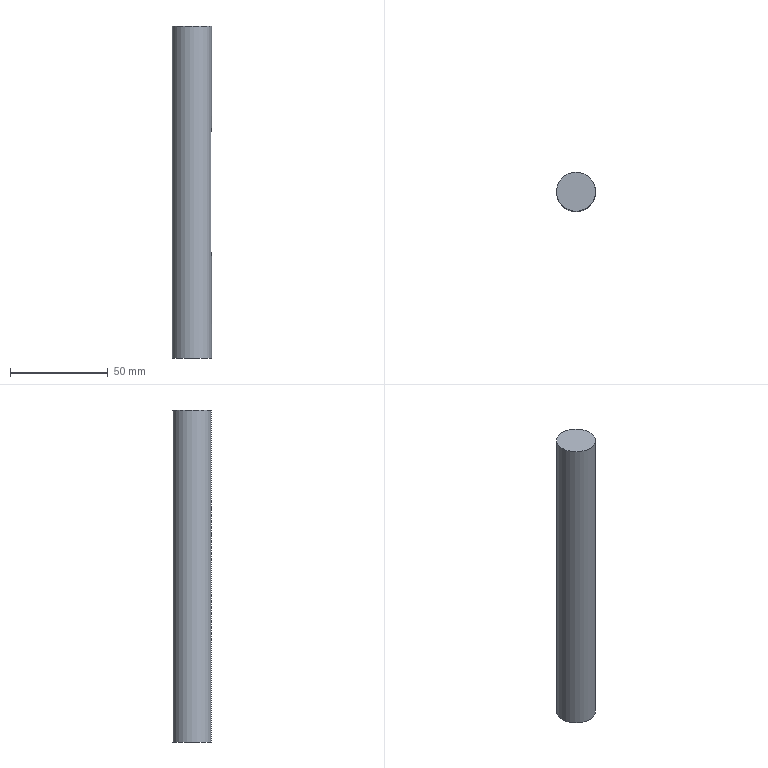Component | NX | CAMSHAFT | 1 solid | 8 faces | box 20 x 20 x 170 mm | volume 52641 mm3 | plane 5 | cylinder 3 | commonest cylinder face diameters 5 x2 20 x1
STEP:
#1=CARTESIAN_POINT('',(0.,0.,0.));
#2=DIRECTION('',(0.,0.,1.));
#3=DIRECTION('',(1.,0.,0.));
#4=AXIS2_PLACEMENT_3D('',#1,#2,#3);
#5=CARTESIAN_POINT('',(10.,0.,90.));
#6=VERTEX_POINT('',#5);
#7=CARTESIAN_POINT('',(0.,0.,90.));
#8=DIRECTION('',(0.,0.,1.));
#9=DIRECTION('',(1.,0.,0.));
#10=AXIS2_PLACEMENT_3D('',#7,#8,#9);
#11=CIRCLE('',#10,10.);
#12=CARTESIAN_POINT('',(0.,0.,260.));
#13=DIRECTION('',(0.,0.,-1.));
#14=DIRECTION('',(-1.,0.,0.));
#15=AXIS2_PLACEMENT_3D('',#12,#13,#14);
#16=CYLINDRICAL_SURFACE('',#15,10.);
#17=CARTESIAN_POINT('',(9.425,170.));
#18=DIRECTION('',(-1.,0.));
#19=VECTOR('',#18,1.);
#20=LINE('',#17,#19);
#21=(GEOMETRIC_REPRESENTATION_CONTEXT(2)PARAMETRIC_REPRESENTATION_CONTEXT()REPRESENTATION_CONTEXT('',''));
#22=DEFINITIONAL_REPRESENTATION('',(#20),#21);
#23=PCURVE('',#16,#22);
#24=CARTESIAN_POINT('',(0.,0.,90.));
#25=DIRECTION('',(0.,0.,1.));
#26=DIRECTION('',(1.,0.,0.));
#27=AXIS2_PLACEMENT_3D('',#24,#25,#26);
#28=PLANE('',#27);
#29=CARTESIAN_POINT('',(0.,0.));
#30=DIRECTION('',(1.,0.));
#31=AXIS2_PLACEMENT_2D('',#29,#30);
#32=CIRCLE('',#31,10.);
#33=(GEOMETRIC_REPRESENTATION_CONTEXT(2)PARAMETRIC_REPRESENTATION_CONTEXT()REPRESENTATION_CONTEXT('',''));
#34=DEFINITIONAL_REPRESENTATION('',(#32),#33);
#35=PCURVE('',#28,#34);
#36=SURFACE_CURVE('',#11,(#23,#35),.PCURVE_S1.);
#37=EDGE_CURVE('',#6,#6,#36,.T.);
#38=ORIENTED_EDGE('',*,*,#37,.T.);
#39=CARTESIAN_POINT('',(10.,0.,142.5));
#40=VERTEX_POINT('',#39);
#41=CARTESIAN_POINT('',(10.,0.,142.5));
#42=CARTESIAN_POINT('',(10.,0.,90.));
#43=B_SPLINE_CURVE_WITH_KNOTS('',1,(#41,#42),.UNSPECIFIED.,.F.,.F.,(2,2),(117.5,170.),.PIECEWISE_BEZIER_KNOTS.);
#44=CARTESIAN_POINT('',(3.142,0.));
#45=DIRECTION('',(0.,1.));
#46=VECTOR('',#45,1.);
#47=LINE('',#44,#46);
#48=(GEOMETRIC_REPRESENTATION_CONTEXT(2)PARAMETRIC_REPRESENTATION_CONTEXT()REPRESENTATION_CONTEXT('',''));
#49=DEFINITIONAL_REPRESENTATION('',(#47),#48);
#50=PCURVE('',#16,#49);
#51=CARTESIAN_POINT('',(9.425,0.));
#52=DIRECTION('',(0.,1.));
#53=VECTOR('',#52,1.);
#54=LINE('',#51,#53);
#55=(GEOMETRIC_REPRESENTATION_CONTEXT(2)PARAMETRIC_REPRESENTATION_CONTEXT()REPRESENTATION_CONTEXT('',''));
#56=DEFINITIONAL_REPRESENTATION('',(#54),#55);
#57=PCURVE('',#16,#56);
#58=SEAM_CURVE('',#43,(#50,#57),.PCURVE_S1.);
#59=EDGE_CURVE('',#40,#6,#58,.T.);
#60=ORIENTED_EDGE('',*,*,#59,.F.);
#61=CARTESIAN_POINT('',(9.682,-2.5,145.));
#62=VERTEX_POINT('',#61);
#63=CARTESIAN_POINT('',(9.682,-2.5,145.));
#64=CARTESIAN_POINT('',(9.682,-2.5,144.725));
#65=CARTESIAN_POINT('',(9.695,-2.453,144.446));
#66=CARTESIAN_POINT('',(9.717,-2.364,144.187));
#67=CARTESIAN_POINT('',(9.738,-2.275,143.928));
#68=CARTESIAN_POINT('',(9.769,-2.142,143.682));
#69=CARTESIAN_POINT('',(9.803,-1.974,143.466));
#70=CARTESIAN_POINT('',(9.838,-1.804,143.247));
#71=CARTESIAN_POINT('',(9.875,-1.594,143.054));
#72=CARTESIAN_POINT('',(9.907,-1.36,142.902));
#73=CARTESIAN_POINT('',(9.94,-1.123,142.749));
#74=CARTESIAN_POINT('',(9.967,-0.8559,142.634));
#75=CARTESIAN_POINT('',(9.983,-0.5801,142.568));
#76=CARTESIAN_POINT('',(9.999,-0.31,142.504));
#77=CARTESIAN_POINT('',(10.004,-0.02421,142.485));
#78=CARTESIAN_POINT('',(9.997,0.2525,142.513));
#79=CARTESIAN_POINT('',(9.99,0.523,142.54));
#80=CARTESIAN_POINT('',(9.972,0.7923,142.613));
#81=CARTESIAN_POINT('',(9.946,1.039,142.726));
#82=CARTESIAN_POINT('',(9.92,1.287,142.84));
#83=CARTESIAN_POINT('',(9.886,1.519,142.996));
#84=CARTESIAN_POINT('',(9.851,1.717,143.183));
#85=CARTESIAN_POINT('',(9.816,1.921,143.375));
#86=CARTESIAN_POINT('',(9.779,2.094,143.605));
#87=CARTESIAN_POINT('',(9.75,2.222,143.854));
#88=CARTESIAN_POINT('',(9.721,2.351,144.105));
#89=CARTESIAN_POINT('',(9.698,2.439,144.382));
#90=CARTESIAN_POINT('',(9.688,2.477,144.663));
#91=CARTESIAN_POINT('',(9.684,2.492,144.774));
#92=CARTESIAN_POINT('',(9.682,2.5,144.887));
#93=CARTESIAN_POINT('',(9.682,2.5,145.));
#94=B_SPLINE_CURVE_WITH_KNOTS('',3,(#63,#64,#65,#66,#67,#68,#69,#70,#71,#72,#73,#74,#75,#76,#77,#78,#79,#80,#81,#82,#83,#84,#85,#86,#87,#88,#89,#90,#91,#92,#93),.UNSPECIFIED.,.F.,.F.,(4,3,3,3,3,3,3,3,3,3,4),(0.,0.1051,0.2101,0.3172,0.4259,0.5323,0.6363,0.7412,0.849,0.9574,1.),.UNSPECIFIED.);
#95=CARTESIAN_POINT('',(3.394,115.));
#96=CARTESIAN_POINT('',(3.394,115.059));
#97=CARTESIAN_POINT('',(3.394,115.179));
#98=CARTESIAN_POINT('',(3.392,115.357));
#99=CARTESIAN_POINT('',(3.389,115.534));
#100=CARTESIAN_POINT('',(3.384,115.707));
#101=CARTESIAN_POINT('',(3.378,115.876));
#102=CARTESIAN_POINT('',(3.371,116.041));
#103=CARTESIAN_POINT('',(3.363,116.201));
#104=CARTESIAN_POINT('',(3.354,116.354));
#105=CARTESIAN_POINT('',(3.343,116.5));
#106=CARTESIAN_POINT('',(3.332,116.638));
#107=CARTESIAN_POINT('',(3.319,116.769));
#108=CARTESIAN_POINT('',(3.306,116.89));
#109=CARTESIAN_POINT('',(3.292,117.002));
#110=CARTESIAN_POINT('',(3.277,117.104));
#111=CARTESIAN_POINT('',(3.262,117.194));
#112=CARTESIAN_POINT('',(3.246,117.274));
#113=CARTESIAN_POINT('',(3.229,117.343));
#114=CARTESIAN_POINT('',(3.212,117.4));
#115=CARTESIAN_POINT('',(3.195,117.444));
#116=CARTESIAN_POINT('',(3.178,117.476));
#117=CARTESIAN_POINT('',(3.16,117.495));
#118=CARTESIAN_POINT('',(3.142,117.502));
#119=CARTESIAN_POINT('',(3.124,117.496));
#120=CARTESIAN_POINT('',(3.106,117.477));
#121=CARTESIAN_POINT('',(3.088,117.445));
#122=CARTESIAN_POINT('',(3.071,117.4));
#123=CARTESIAN_POINT('',(3.054,117.344));
#124=CARTESIAN_POINT('',(3.037,117.276));
#125=CARTESIAN_POINT('',(3.021,117.196));
#126=CARTESIAN_POINT('',(3.006,117.105));
#127=CARTESIAN_POINT('',(2.991,117.003));
#128=CARTESIAN_POINT('',(2.977,116.891));
#129=CARTESIAN_POINT('',(2.964,116.771));
#130=CARTESIAN_POINT('',(2.952,116.64));
#131=CARTESIAN_POINT('',(2.94,116.502));
#132=CARTESIAN_POINT('',(2.93,116.355));
#133=CARTESIAN_POINT('',(2.92,116.202));
#134=CARTESIAN_POINT('',(2.912,116.044));
#135=CARTESIAN_POINT('',(2.905,115.879));
#136=CARTESIAN_POINT('',(2.899,115.709));
#137=CARTESIAN_POINT('',(2.895,115.535));
#138=CARTESIAN_POINT('',(2.891,115.36));
#139=CARTESIAN_POINT('',(2.889,115.181));
#140=CARTESIAN_POINT('',(2.889,115.06));
#141=CARTESIAN_POINT('',(2.889,115.));
#142=B_SPLINE_CURVE_WITH_KNOTS('',3,(#95,#96,#97,#98,#99,#100,#101,#102,#103,#104,#105,#106,#107,#108,#109,#110,#111,#112,#113,#114,#115,#116,#117,#118,#119,#120,#121,#122,#123,#124,#125,#126,#127,#128,#129,#130,#131,#132,#133,#134,#135,#136,#137,#138,#139,#140,#141),.UNSPECIFIED.,.F.,.F.,(4,1,1,1,1,1,1,1,1,1,1,1,1,1,1,1,1,1,1,1,1,1,1,1,1,1,1,1,1,1,1,1,1,1,1,1,1,1,1,1,1,1,1,1,4),(0.,0.02273,0.04545,0.06818,0.09091,0.1136,0.1364,0.1591,0.1818,0.2045,0.2273,0.25,0.2727,0.2955,0.3182,0.3409,0.3636,0.3864,0.4091,0.4318,0.4545,0.4773,0.5,0.5227,0.5455,0.5682,0.5909,0.6136,0.6364,0.6591,0.6818,0.7045,0.7273,0.75,0.7727,0.7955,0.8182,0.8409,0.8636,0.8864,0.9091,0.9318,0.9545,0.9773,1.),.QUASI_UNIFORM_KNOTS.);
#143=(GEOMETRIC_REPRESENTATION_CONTEXT(2)PARAMETRIC_REPRESENTATION_CONTEXT()REPRESENTATION_CONTEXT('',''));
#144=DEFINITIONAL_REPRESENTATION('',(#142),#143);
#145=PCURVE('',#16,#144);
#146=CARTESIAN_POINT('',(32.,0.,145.));
#147=DIRECTION('',(-1.,0.,0.));
#148=DIRECTION('',(0.,0.,1.));
#149=AXIS2_PLACEMENT_3D('',#146,#147,#148);
#150=CYLINDRICAL_SURFACE('',#149,2.5);
#151=CARTESIAN_POINT('',(4.712,22.318));
#152=CARTESIAN_POINT('',(3.142,22.));
#153=B_SPLINE_CURVE_WITH_KNOTS('',1,(#151,#152),.UNSPECIFIED.,.F.,.F.,(2,2),(0.,0.5001),.PIECEWISE_BEZIER_KNOTS.);
#154=(GEOMETRIC_REPRESENTATION_CONTEXT(2)PARAMETRIC_REPRESENTATION_CONTEXT()REPRESENTATION_CONTEXT('',''));
#155=DEFINITIONAL_REPRESENTATION('',(#153),#154);
#156=PCURVE('',#150,#155);
#157=SURFACE_CURVE('',#94,(#145,#156),.PCURVE_S1.);
#158=EDGE_CURVE('',#62,#40,#157,.T.);
#159=ORIENTED_EDGE('',*,*,#158,.F.);
#160=CARTESIAN_POINT('',(9.682,-2.5,205.));
#161=VERTEX_POINT('',#160);
#162=CARTESIAN_POINT('',(9.682,-2.5,260.));
#163=DIRECTION('',(0.,0.,-1.));
#164=VECTOR('',#163,1.);
#165=LINE('',#162,#164);
#166=CARTESIAN_POINT('',(3.394,0.));
#167=DIRECTION('',(0.,1.));
#168=VECTOR('',#167,1.);
#169=LINE('',#166,#168);
#170=(GEOMETRIC_REPRESENTATION_CONTEXT(2)PARAMETRIC_REPRESENTATION_CONTEXT()REPRESENTATION_CONTEXT('',''));
#171=DEFINITIONAL_REPRESENTATION('',(#169),#170);
#172=PCURVE('',#16,#171);
#173=CARTESIAN_POINT('',(32.,-2.5,205.));
#174=DIRECTION('',(0.,1.,0.));
#175=DIRECTION('',(0.,0.,1.));
#176=AXIS2_PLACEMENT_3D('',#173,#174,#175);
#177=PLANE('',#176);
#178=CARTESIAN_POINT('',(55.,-22.318));
#179=DIRECTION('',(-1.,0.));
#180=VECTOR('',#179,1.);
#181=LINE('',#178,#180);
#182=(GEOMETRIC_REPRESENTATION_CONTEXT(2)PARAMETRIC_REPRESENTATION_CONTEXT()REPRESENTATION_CONTEXT('',''));
#183=DEFINITIONAL_REPRESENTATION('',(#181),#182);
#184=PCURVE('',#177,#183);
#185=SURFACE_CURVE('',#165,(#172,#184),.PCURVE_S1.);
#186=EDGE_CURVE('',#161,#62,#185,.T.);
#187=ORIENTED_EDGE('',*,*,#186,.F.);
#188=CARTESIAN_POINT('',(10.,0.,207.5));
#189=VERTEX_POINT('',#188);
#190=CARTESIAN_POINT('',(9.682,2.5,205.));
#191=CARTESIAN_POINT('',(9.682,2.5,205.275));
#192=CARTESIAN_POINT('',(9.695,2.453,205.554));
#193=CARTESIAN_POINT('',(9.717,2.364,205.813));
#194=CARTESIAN_POINT('',(9.738,2.275,206.072));
#195=CARTESIAN_POINT('',(9.769,2.142,206.318));
#196=CARTESIAN_POINT('',(9.803,1.974,206.534));
#197=CARTESIAN_POINT('',(9.838,1.804,206.753));
#198=CARTESIAN_POINT('',(9.875,1.594,206.946));
#199=CARTESIAN_POINT('',(9.907,1.36,207.098));
#200=CARTESIAN_POINT('',(9.94,1.123,207.251));
#201=CARTESIAN_POINT('',(9.967,0.8559,207.366));
#202=CARTESIAN_POINT('',(9.983,0.5801,207.432));
#203=CARTESIAN_POINT('',(9.999,0.31,207.496));
#204=CARTESIAN_POINT('',(10.004,0.02421,207.515));
#205=CARTESIAN_POINT('',(9.997,-0.2525,207.487));
#206=CARTESIAN_POINT('',(9.99,-0.523,207.46));
#207=CARTESIAN_POINT('',(9.972,-0.7923,207.387));
#208=CARTESIAN_POINT('',(9.946,-1.039,207.274));
#209=CARTESIAN_POINT('',(9.92,-1.287,207.16));
#210=CARTESIAN_POINT('',(9.886,-1.519,207.004));
#211=CARTESIAN_POINT('',(9.851,-1.717,206.817));
#212=CARTESIAN_POINT('',(9.816,-1.921,206.625));
#213=CARTESIAN_POINT('',(9.779,-2.094,206.395));
#214=CARTESIAN_POINT('',(9.75,-2.222,206.146));
#215=CARTESIAN_POINT('',(9.721,-2.351,205.895));
#216=CARTESIAN_POINT('',(9.698,-2.439,205.618));
#217=CARTESIAN_POINT('',(9.688,-2.477,205.337));
#218=CARTESIAN_POINT('',(9.684,-2.492,205.226));
#219=CARTESIAN_POINT('',(9.682,-2.5,205.113));
#220=CARTESIAN_POINT('',(9.682,-2.5,205.));
#221=B_SPLINE_CURVE_WITH_KNOTS('',3,(#190,#191,#192,#193,#194,#195,#196,#197,#198,#199,#200,#201,#202,#203,#204,#205,#206,#207,#208,#209,#210,#211,#212,#213,#214,#215,#216,#217,#218,#219,#220),.UNSPECIFIED.,.F.,.F.,(4,3,3,3,3,3,3,3,3,3,4),(0.,0.1051,0.2101,0.3172,0.4259,0.5323,0.6363,0.7412,0.849,0.9574,1.),.UNSPECIFIED.);
#222=CARTESIAN_POINT('',(2.889,55.));
#223=CARTESIAN_POINT('',(2.889,54.941));
#224=CARTESIAN_POINT('',(2.889,54.821));
#225=CARTESIAN_POINT('',(2.891,54.643));
#226=CARTESIAN_POINT('',(2.895,54.466));
#227=CARTESIAN_POINT('',(2.899,54.293));
#228=CARTESIAN_POINT('',(2.905,54.124));
#229=CARTESIAN_POINT('',(2.912,53.959));
#230=CARTESIAN_POINT('',(2.92,53.799));
#231=CARTESIAN_POINT('',(2.93,53.646));
#232=CARTESIAN_POINT('',(2.94,53.5));
#233=CARTESIAN_POINT('',(2.951,53.362));
#234=CARTESIAN_POINT('',(2.964,53.231));
#235=CARTESIAN_POINT('',(2.977,53.11));
#236=CARTESIAN_POINT('',(2.991,52.998));
#237=CARTESIAN_POINT('',(3.006,52.896));
#238=CARTESIAN_POINT('',(3.021,52.806));
#239=CARTESIAN_POINT('',(3.037,52.726));
#240=CARTESIAN_POINT('',(3.054,52.657));
#241=CARTESIAN_POINT('',(3.071,52.6));
#242=CARTESIAN_POINT('',(3.088,52.556));
#243=CARTESIAN_POINT('',(3.106,52.524));
#244=CARTESIAN_POINT('',(3.124,52.505));
#245=CARTESIAN_POINT('',(3.141,52.498));
#246=CARTESIAN_POINT('',(3.159,52.504));
#247=CARTESIAN_POINT('',(3.177,52.523));
#248=CARTESIAN_POINT('',(3.195,52.555));
#249=CARTESIAN_POINT('',(3.212,52.6));
#250=CARTESIAN_POINT('',(3.229,52.656));
#251=CARTESIAN_POINT('',(3.246,52.724));
#252=CARTESIAN_POINT('',(3.262,52.804));
#253=CARTESIAN_POINT('',(3.277,52.895));
#254=CARTESIAN_POINT('',(3.292,52.997));
#255=CARTESIAN_POINT('',(3.306,53.109));
#256=CARTESIAN_POINT('',(3.319,53.229));
#257=CARTESIAN_POINT('',(3.332,53.36));
#258=CARTESIAN_POINT('',(3.343,53.498));
#259=CARTESIAN_POINT('',(3.353,53.645));
#260=CARTESIAN_POINT('',(3.363,53.798));
#261=CARTESIAN_POINT('',(3.371,53.956));
#262=CARTESIAN_POINT('',(3.378,54.121));
#263=CARTESIAN_POINT('',(3.384,54.291));
#264=CARTESIAN_POINT('',(3.388,54.465));
#265=CARTESIAN_POINT('',(3.392,54.64));
#266=CARTESIAN_POINT('',(3.394,54.819));
#267=CARTESIAN_POINT('',(3.394,54.94));
#268=CARTESIAN_POINT('',(3.394,55.));
#269=B_SPLINE_CURVE_WITH_KNOTS('',3,(#222,#223,#224,#225,#226,#227,#228,#229,#230,#231,#232,#233,#234,#235,#236,#237,#238,#239,#240,#241,#242,#243,#244,#245,#246,#247,#248,#249,#250,#251,#252,#253,#254,#255,#256,#257,#258,#259,#260,#261,#262,#263,#264,#265,#266,#267,#268),.UNSPECIFIED.,.F.,.F.,(4,1,1,1,1,1,1,1,1,1,1,1,1,1,1,1,1,1,1,1,1,1,1,1,1,1,1,1,1,1,1,1,1,1,1,1,1,1,1,1,1,1,1,1,4),(0.,0.02273,0.04545,0.06818,0.09091,0.1136,0.1364,0.1591,0.1818,0.2045,0.2273,0.25,0.2727,0.2955,0.3182,0.3409,0.3636,0.3864,0.4091,0.4318,0.4545,0.4773,0.5,0.5227,0.5455,0.5682,0.5909,0.6136,0.6364,0.6591,0.6818,0.7045,0.7273,0.75,0.7727,0.7955,0.8182,0.8409,0.8636,0.8864,0.9091,0.9318,0.9545,0.9773,1.),.QUASI_UNIFORM_KNOTS.);
#270=(GEOMETRIC_REPRESENTATION_CONTEXT(2)PARAMETRIC_REPRESENTATION_CONTEXT()REPRESENTATION_CONTEXT('',''));
#271=DEFINITIONAL_REPRESENTATION('',(#269),#270);
#272=PCURVE('',#16,#271);
#273=CARTESIAN_POINT('',(32.,0.,205.));
#274=DIRECTION('',(-1.,0.,0.));
#275=DIRECTION('',(0.,0.,1.));
#276=AXIS2_PLACEMENT_3D('',#273,#274,#275);
#277=CYLINDRICAL_SURFACE('',#276,2.5);
#278=CARTESIAN_POINT('',(-0.00000001,22.));
#279=CARTESIAN_POINT('',(-1.571,22.318));
#280=B_SPLINE_CURVE_WITH_KNOTS('',1,(#278,#279),.UNSPECIFIED.,.F.,.F.,(2,2),(0.5001,1.),.PIECEWISE_BEZIER_KNOTS.);
#281=(GEOMETRIC_REPRESENTATION_CONTEXT(2)PARAMETRIC_REPRESENTATION_CONTEXT()REPRESENTATION_CONTEXT('',''));
#282=DEFINITIONAL_REPRESENTATION('',(#280),#281);
#283=PCURVE('',#277,#282);
#284=SURFACE_CURVE('',#221,(#272,#283),.PCURVE_S1.);
#285=EDGE_CURVE('',#189,#161,#284,.T.);
#286=ORIENTED_EDGE('',*,*,#285,.F.);
#287=CARTESIAN_POINT('',(10.,0.,260.));
#288=VERTEX_POINT('',#287);
#289=CARTESIAN_POINT('',(10.,0.,260.));
#290=CARTESIAN_POINT('',(10.,0.,207.5));
#291=B_SPLINE_CURVE_WITH_KNOTS('',1,(#289,#290),.UNSPECIFIED.,.F.,.F.,(2,2),(0.,52.5),.PIECEWISE_BEZIER_KNOTS.);
#292=CARTESIAN_POINT('',(3.142,0.));
#293=DIRECTION('',(0.,1.));
#294=VECTOR('',#293,1.);
#295=LINE('',#292,#294);
#296=(GEOMETRIC_REPRESENTATION_CONTEXT(2)PARAMETRIC_REPRESENTATION_CONTEXT()REPRESENTATION_CONTEXT('',''));
#297=DEFINITIONAL_REPRESENTATION('',(#295),#296);
#298=PCURVE('',#16,#297);
#299=CARTESIAN_POINT('',(9.425,0.));
#300=DIRECTION('',(0.,1.));
#301=VECTOR('',#300,1.);
#302=LINE('',#299,#301);
#303=(GEOMETRIC_REPRESENTATION_CONTEXT(2)PARAMETRIC_REPRESENTATION_CONTEXT()REPRESENTATION_CONTEXT('',''));
#304=DEFINITIONAL_REPRESENTATION('',(#302),#303);
#305=PCURVE('',#16,#304);
#306=SEAM_CURVE('',#291,(#298,#305),.PCURVE_S1.);
#307=EDGE_CURVE('',#288,#189,#306,.T.);
#308=ORIENTED_EDGE('',*,*,#307,.F.);
#309=CARTESIAN_POINT('',(0.,0.,260.));
#310=DIRECTION('',(0.,0.,1.));
#311=DIRECTION('',(1.,0.,0.));
#312=AXIS2_PLACEMENT_3D('',#309,#310,#311);
#313=CIRCLE('',#312,10.);
#314=CARTESIAN_POINT('',(9.425,0.));
#315=DIRECTION('',(-1.,0.));
#316=VECTOR('',#315,1.);
#317=LINE('',#314,#316);
#318=(GEOMETRIC_REPRESENTATION_CONTEXT(2)PARAMETRIC_REPRESENTATION_CONTEXT()REPRESENTATION_CONTEXT('',''));
#319=DEFINITIONAL_REPRESENTATION('',(#317),#318);
#320=PCURVE('',#16,#319);
#321=CARTESIAN_POINT('',(0.,0.,260.));
#322=DIRECTION('',(0.,0.,1.));
#323=DIRECTION('',(1.,0.,0.));
#324=AXIS2_PLACEMENT_3D('',#321,#322,#323);
#325=PLANE('',#324);
#326=CARTESIAN_POINT('',(0.,0.));
#327=DIRECTION('',(1.,0.));
#328=AXIS2_PLACEMENT_2D('',#326,#327);
#329=CIRCLE('',#328,10.);
#330=(GEOMETRIC_REPRESENTATION_CONTEXT(2)PARAMETRIC_REPRESENTATION_CONTEXT()REPRESENTATION_CONTEXT('',''));
#331=DEFINITIONAL_REPRESENTATION('',(#329),#330);
#332=PCURVE('',#325,#331);
#333=SURFACE_CURVE('',#313,(#320,#332),.PCURVE_S1.);
#334=EDGE_CURVE('',#288,#288,#333,.T.);
#335=ORIENTED_EDGE('',*,*,#334,.F.);
#336=ORIENTED_EDGE('',*,*,#307,.T.);
#337=CARTESIAN_POINT('',(9.682,2.5,205.));
#338=VERTEX_POINT('',#337);
#339=CARTESIAN_POINT('',(9.682,2.5,205.));
#340=CARTESIAN_POINT('',(9.682,2.5,205.275));
#341=CARTESIAN_POINT('',(9.695,2.453,205.554));
#342=CARTESIAN_POINT('',(9.717,2.364,205.813));
#343=CARTESIAN_POINT('',(9.738,2.275,206.072));
#344=CARTESIAN_POINT('',(9.769,2.142,206.318));
#345=CARTESIAN_POINT('',(9.803,1.974,206.534));
#346=CARTESIAN_POINT('',(9.838,1.804,206.753));
#347=CARTESIAN_POINT('',(9.875,1.594,206.946));
#348=CARTESIAN_POINT('',(9.907,1.36,207.098));
#349=CARTESIAN_POINT('',(9.94,1.123,207.251));
#350=CARTESIAN_POINT('',(9.967,0.8559,207.366));
#351=CARTESIAN_POINT('',(9.983,0.5801,207.432));
#352=CARTESIAN_POINT('',(9.999,0.31,207.496));
#353=CARTESIAN_POINT('',(10.004,0.02421,207.515));
#354=CARTESIAN_POINT('',(9.997,-0.2525,207.487));
#355=CARTESIAN_POINT('',(9.99,-0.523,207.46));
#356=CARTESIAN_POINT('',(9.972,-0.7923,207.387));
#357=CARTESIAN_POINT('',(9.946,-1.039,207.274));
#358=CARTESIAN_POINT('',(9.92,-1.287,207.16));
#359=CARTESIAN_POINT('',(9.886,-1.519,207.004));
#360=CARTESIAN_POINT('',(9.851,-1.717,206.817));
#361=CARTESIAN_POINT('',(9.816,-1.921,206.625));
#362=CARTESIAN_POINT('',(9.779,-2.094,206.395));
#363=CARTESIAN_POINT('',(9.75,-2.222,206.146));
#364=CARTESIAN_POINT('',(9.721,-2.351,205.895));
#365=CARTESIAN_POINT('',(9.698,-2.439,205.618));
#366=CARTESIAN_POINT('',(9.688,-2.477,205.337));
#367=CARTESIAN_POINT('',(9.684,-2.492,205.226));
#368=CARTESIAN_POINT('',(9.682,-2.5,205.113));
#369=CARTESIAN_POINT('',(9.682,-2.5,205.));
#370=B_SPLINE_CURVE_WITH_KNOTS('',3,(#339,#340,#341,#342,#343,#344,#345,#346,#347,#348,#349,#350,#351,#352,#353,#354,#355,#356,#357,#358,#359,#360,#361,#362,#363,#364,#365,#366,#367,#368,#369),.UNSPECIFIED.,.F.,.F.,(4,3,3,3,3,3,3,3,3,3,4),(0.,0.1051,0.2101,0.3172,0.4259,0.5323,0.6363,0.7412,0.849,0.9574,1.),.UNSPECIFIED.);
#371=CARTESIAN_POINT('',(9.172,55.));
#372=CARTESIAN_POINT('',(9.172,54.941));
#373=CARTESIAN_POINT('',(9.173,54.821));
#374=CARTESIAN_POINT('',(9.175,54.643));
#375=CARTESIAN_POINT('',(9.178,54.466));
#376=CARTESIAN_POINT('',(9.182,54.293));
#377=CARTESIAN_POINT('',(9.188,54.124));
#378=CARTESIAN_POINT('',(9.195,53.959));
#379=CARTESIAN_POINT('',(9.203,53.799));
#380=CARTESIAN_POINT('',(9.213,53.646));
#381=CARTESIAN_POINT('',(9.223,53.5));
#382=CARTESIAN_POINT('',(9.235,53.362));
#383=CARTESIAN_POINT('',(9.247,53.231));
#384=CARTESIAN_POINT('',(9.26,53.11));
#385=CARTESIAN_POINT('',(9.274,52.998));
#386=CARTESIAN_POINT('',(9.289,52.896));
#387=CARTESIAN_POINT('',(9.304,52.806));
#388=CARTESIAN_POINT('',(9.32,52.726));
#389=CARTESIAN_POINT('',(9.337,52.657));
#390=CARTESIAN_POINT('',(9.354,52.6));
#391=CARTESIAN_POINT('',(9.371,52.556));
#392=CARTESIAN_POINT('',(9.389,52.524));
#393=CARTESIAN_POINT('',(9.407,52.505));
#394=CARTESIAN_POINT('',(9.425,52.498));
#395=CARTESIAN_POINT('',(9.443,52.504));
#396=CARTESIAN_POINT('',(9.46,52.523));
#397=CARTESIAN_POINT('',(9.478,52.555));
#398=CARTESIAN_POINT('',(9.495,52.6));
#399=CARTESIAN_POINT('',(9.512,52.656));
#400=CARTESIAN_POINT('',(9.529,52.724));
#401=CARTESIAN_POINT('',(9.545,52.804));
#402=CARTESIAN_POINT('',(9.56,52.895));
#403=CARTESIAN_POINT('',(9.575,52.997));
#404=CARTESIAN_POINT('',(9.589,53.109));
#405=CARTESIAN_POINT('',(9.602,53.229));
#406=CARTESIAN_POINT('',(9.615,53.36));
#407=CARTESIAN_POINT('',(9.626,53.498));
#408=CARTESIAN_POINT('',(9.637,53.645));
#409=CARTESIAN_POINT('',(9.646,53.798));
#410=CARTESIAN_POINT('',(9.654,53.956));
#411=CARTESIAN_POINT('',(9.661,54.121));
#412=CARTESIAN_POINT('',(9.667,54.291));
#413=CARTESIAN_POINT('',(9.672,54.465));
#414=CARTESIAN_POINT('',(9.675,54.64));
#415=CARTESIAN_POINT('',(9.677,54.819));
#416=CARTESIAN_POINT('',(9.677,54.94));
#417=CARTESIAN_POINT('',(9.677,55.));
#418=B_SPLINE_CURVE_WITH_KNOTS('',3,(#371,#372,#373,#374,#375,#376,#377,#378,#379,#380,#381,#382,#383,#384,#385,#386,#387,#388,#389,#390,#391,#392,#393,#394,#395,#396,#397,#398,#399,#400,#401,#402,#403,#404,#405,#406,#407,#408,#409,#410,#411,#412,#413,#414,#415,#416,#417),.UNSPECIFIED.,.F.,.F.,(4,1,1,1,1,1,1,1,1,1,1,1,1,1,1,1,1,1,1,1,1,1,1,1,1,1,1,1,1,1,1,1,1,1,1,1,1,1,1,1,1,1,1,1,4),(0.,0.02273,0.04545,0.06818,0.09091,0.1136,0.1364,0.1591,0.1818,0.2045,0.2273,0.25,0.2727,0.2955,0.3182,0.3409,0.3636,0.3864,0.4091,0.4318,0.4545,0.4773,0.5,0.5227,0.5455,0.5682,0.5909,0.6136,0.6364,0.6591,0.6818,0.7045,0.7273,0.75,0.7727,0.7955,0.8182,0.8409,0.8636,0.8864,0.9091,0.9318,0.9545,0.9773,1.),.QUASI_UNIFORM_KNOTS.);
#419=(GEOMETRIC_REPRESENTATION_CONTEXT(2)PARAMETRIC_REPRESENTATION_CONTEXT()REPRESENTATION_CONTEXT('',''));
#420=DEFINITIONAL_REPRESENTATION('',(#418),#419);
#421=PCURVE('',#16,#420);
#422=CARTESIAN_POINT('',(1.571,22.318));
#423=CARTESIAN_POINT('',(-0.00000001,22.));
#424=B_SPLINE_CURVE_WITH_KNOTS('',1,(#422,#423),.UNSPECIFIED.,.F.,.F.,(2,2),(0.,0.5001),.PIECEWISE_BEZIER_KNOTS.);
#425=(GEOMETRIC_REPRESENTATION_CONTEXT(2)PARAMETRIC_REPRESENTATION_CONTEXT()REPRESENTATION_CONTEXT('',''));
#426=DEFINITIONAL_REPRESENTATION('',(#424),#425);
#427=PCURVE('',#277,#426);
#428=SURFACE_CURVE('',#370,(#421,#427),.PCURVE_S1.);
#429=EDGE_CURVE('',#338,#189,#428,.T.);
#430=ORIENTED_EDGE('',*,*,#429,.F.);
#431=CARTESIAN_POINT('',(9.682,2.5,145.));
#432=VERTEX_POINT('',#431);
#433=CARTESIAN_POINT('',(9.682,2.5,260.));
#434=DIRECTION('',(0.,0.,1.));
#435=VECTOR('',#434,1.);
#436=LINE('',#433,#435);
#437=CARTESIAN_POINT('',(9.172,0.));
#438=DIRECTION('',(0.,-1.));
#439=VECTOR('',#438,1.);
#440=LINE('',#437,#439);
#441=(GEOMETRIC_REPRESENTATION_CONTEXT(2)PARAMETRIC_REPRESENTATION_CONTEXT()REPRESENTATION_CONTEXT('',''));
#442=DEFINITIONAL_REPRESENTATION('',(#440),#441);
#443=PCURVE('',#16,#442);
#444=CARTESIAN_POINT('',(32.,2.5,145.));
#445=DIRECTION('',(0.,-1.,0.));
#446=DIRECTION('',(0.,0.,-1.));
#447=AXIS2_PLACEMENT_3D('',#444,#445,#446);
#448=PLANE('',#447);
#449=CARTESIAN_POINT('',(-115.,-22.318));
#450=DIRECTION('',(-1.,0.));
#451=VECTOR('',#450,1.);
#452=LINE('',#449,#451);
#453=(GEOMETRIC_REPRESENTATION_CONTEXT(2)PARAMETRIC_REPRESENTATION_CONTEXT()REPRESENTATION_CONTEXT('',''));
#454=DEFINITIONAL_REPRESENTATION('',(#452),#453);
#455=PCURVE('',#448,#454);
#456=SURFACE_CURVE('',#436,(#443,#455),.PCURVE_S1.);
#457=EDGE_CURVE('',#432,#338,#456,.T.);
#458=ORIENTED_EDGE('',*,*,#457,.F.);
#459=CARTESIAN_POINT('',(9.682,-2.5,145.));
#460=CARTESIAN_POINT('',(9.682,-2.5,144.725));
#461=CARTESIAN_POINT('',(9.695,-2.453,144.446));
#462=CARTESIAN_POINT('',(9.717,-2.364,144.187));
#463=CARTESIAN_POINT('',(9.738,-2.275,143.928));
#464=CARTESIAN_POINT('',(9.769,-2.142,143.682));
#465=CARTESIAN_POINT('',(9.803,-1.974,143.466));
#466=CARTESIAN_POINT('',(9.838,-1.804,143.247));
#467=CARTESIAN_POINT('',(9.875,-1.594,143.054));
#468=CARTESIAN_POINT('',(9.907,-1.36,142.902));
#469=CARTESIAN_POINT('',(9.94,-1.123,142.749));
#470=CARTESIAN_POINT('',(9.967,-0.8559,142.634));
#471=CARTESIAN_POINT('',(9.983,-0.5801,142.568));
#472=CARTESIAN_POINT('',(9.999,-0.31,142.504));
#473=CARTESIAN_POINT('',(10.004,-0.02421,142.485));
#474=CARTESIAN_POINT('',(9.997,0.2525,142.513));
#475=CARTESIAN_POINT('',(9.99,0.523,142.54));
#476=CARTESIAN_POINT('',(9.972,0.7923,142.613));
#477=CARTESIAN_POINT('',(9.946,1.039,142.726));
#478=CARTESIAN_POINT('',(9.92,1.287,142.84));
#479=CARTESIAN_POINT('',(9.886,1.519,142.996));
#480=CARTESIAN_POINT('',(9.851,1.717,143.183));
#481=CARTESIAN_POINT('',(9.816,1.921,143.375));
#482=CARTESIAN_POINT('',(9.779,2.094,143.605));
#483=CARTESIAN_POINT('',(9.75,2.222,143.854));
#484=CARTESIAN_POINT('',(9.721,2.351,144.105));
#485=CARTESIAN_POINT('',(9.698,2.439,144.382));
#486=CARTESIAN_POINT('',(9.688,2.477,144.663));
#487=CARTESIAN_POINT('',(9.684,2.492,144.774));
#488=CARTESIAN_POINT('',(9.682,2.5,144.887));
#489=CARTESIAN_POINT('',(9.682,2.5,145.));
#490=B_SPLINE_CURVE_WITH_KNOTS('',3,(#459,#460,#461,#462,#463,#464,#465,#466,#467,#468,#469,#470,#471,#472,#473,#474,#475,#476,#477,#478,#479,#480,#481,#482,#483,#484,#485,#486,#487,#488,#489),.UNSPECIFIED.,.F.,.F.,(4,3,3,3,3,3,3,3,3,3,4),(0.,0.1051,0.2101,0.3172,0.4259,0.5323,0.6363,0.7412,0.849,0.9574,1.),.UNSPECIFIED.);
#491=CARTESIAN_POINT('',(9.677,115.));
#492=CARTESIAN_POINT('',(9.677,115.059));
#493=CARTESIAN_POINT('',(9.677,115.179));
#494=CARTESIAN_POINT('',(9.675,115.357));
#495=CARTESIAN_POINT('',(9.672,115.534));
#496=CARTESIAN_POINT('',(9.667,115.707));
#497=CARTESIAN_POINT('',(9.661,115.876));
#498=CARTESIAN_POINT('',(9.654,116.041));
#499=CARTESIAN_POINT('',(9.646,116.201));
#500=CARTESIAN_POINT('',(9.637,116.354));
#501=CARTESIAN_POINT('',(9.626,116.5));
#502=CARTESIAN_POINT('',(9.615,116.638));
#503=CARTESIAN_POINT('',(9.603,116.769));
#504=CARTESIAN_POINT('',(9.589,116.89));
#505=CARTESIAN_POINT('',(9.575,117.002));
#506=CARTESIAN_POINT('',(9.561,117.104));
#507=CARTESIAN_POINT('',(9.545,117.194));
#508=CARTESIAN_POINT('',(9.529,117.274));
#509=CARTESIAN_POINT('',(9.513,117.343));
#510=CARTESIAN_POINT('',(9.496,117.4));
#511=CARTESIAN_POINT('',(9.478,117.444));
#512=CARTESIAN_POINT('',(9.461,117.476));
#513=CARTESIAN_POINT('',(9.443,117.495));
#514=CARTESIAN_POINT('',(9.425,117.502));
#515=CARTESIAN_POINT('',(9.407,117.496));
#516=CARTESIAN_POINT('',(9.389,117.477));
#517=CARTESIAN_POINT('',(9.372,117.445));
#518=CARTESIAN_POINT('',(9.354,117.4));
#519=CARTESIAN_POINT('',(9.337,117.344));
#520=CARTESIAN_POINT('',(9.321,117.276));
#521=CARTESIAN_POINT('',(9.305,117.196));
#522=CARTESIAN_POINT('',(9.289,117.105));
#523=CARTESIAN_POINT('',(9.274,117.003));
#524=CARTESIAN_POINT('',(9.26,116.891));
#525=CARTESIAN_POINT('',(9.247,116.771));
#526=CARTESIAN_POINT('',(9.235,116.64));
#527=CARTESIAN_POINT('',(9.223,116.502));
#528=CARTESIAN_POINT('',(9.213,116.355));
#529=CARTESIAN_POINT('',(9.204,116.202));
#530=CARTESIAN_POINT('',(9.195,116.044));
#531=CARTESIAN_POINT('',(9.188,115.879));
#532=CARTESIAN_POINT('',(9.182,115.709));
#533=CARTESIAN_POINT('',(9.178,115.535));
#534=CARTESIAN_POINT('',(9.175,115.36));
#535=CARTESIAN_POINT('',(9.173,115.181));
#536=CARTESIAN_POINT('',(9.172,115.06));
#537=CARTESIAN_POINT('',(9.172,115.));
#538=B_SPLINE_CURVE_WITH_KNOTS('',3,(#491,#492,#493,#494,#495,#496,#497,#498,#499,#500,#501,#502,#503,#504,#505,#506,#507,#508,#509,#510,#511,#512,#513,#514,#515,#516,#517,#518,#519,#520,#521,#522,#523,#524,#525,#526,#527,#528,#529,#530,#531,#532,#533,#534,#535,#536,#537),.UNSPECIFIED.,.F.,.F.,(4,1,1,1,1,1,1,1,1,1,1,1,1,1,1,1,1,1,1,1,1,1,1,1,1,1,1,1,1,1,1,1,1,1,1,1,1,1,1,1,1,1,1,1,4),(0.,0.02273,0.04545,0.06818,0.09091,0.1136,0.1364,0.1591,0.1818,0.2045,0.2273,0.25,0.2727,0.2955,0.3182,0.3409,0.3636,0.3864,0.4091,0.4318,0.4545,0.4773,0.5,0.5227,0.5455,0.5682,0.5909,0.6136,0.6364,0.6591,0.6818,0.7045,0.7273,0.75,0.7727,0.7955,0.8182,0.8409,0.8636,0.8864,0.9091,0.9318,0.9545,0.9773,1.),.QUASI_UNIFORM_KNOTS.);
#539=(GEOMETRIC_REPRESENTATION_CONTEXT(2)PARAMETRIC_REPRESENTATION_CONTEXT()REPRESENTATION_CONTEXT('',''));
#540=DEFINITIONAL_REPRESENTATION('',(#538),#539);
#541=PCURVE('',#16,#540);
#542=CARTESIAN_POINT('',(3.142,22.));
#543=CARTESIAN_POINT('',(1.571,22.318));
#544=B_SPLINE_CURVE_WITH_KNOTS('',1,(#542,#543),.UNSPECIFIED.,.F.,.F.,(2,2),(0.5001,1.),.PIECEWISE_BEZIER_KNOTS.);
#545=(GEOMETRIC_REPRESENTATION_CONTEXT(2)PARAMETRIC_REPRESENTATION_CONTEXT()REPRESENTATION_CONTEXT('',''));
#546=DEFINITIONAL_REPRESENTATION('',(#544),#545);
#547=PCURVE('',#150,#546);
#548=SURFACE_CURVE('',#490,(#541,#547),.PCURVE_S1.);
#549=EDGE_CURVE('',#40,#432,#548,.T.);
#550=ORIENTED_EDGE('',*,*,#549,.F.);
#551=ORIENTED_EDGE('',*,*,#59,.T.);
#552=EDGE_LOOP('',(#38,#60,#159,#187,#286,#308,#335,#336,#430,#458,#550,#551));
#553=FACE_BOUND('',#552,.T.);
#554=ADVANCED_FACE('',(#553),#16,.T.);
#555=ORIENTED_EDGE('',*,*,#334,.T.);
#556=EDGE_LOOP('',(#555));
#557=FACE_BOUND('',#556,.T.);
#558=ADVANCED_FACE('',(#557),#325,.T.);
#559=ORIENTED_EDGE('',*,*,#37,.F.);
#560=EDGE_LOOP('',(#559));
#561=FACE_BOUND('',#560,.T.);
#562=ADVANCED_FACE('',(#561),#28,.F.);
#563=ORIENTED_EDGE('',*,*,#186,.T.);
#564=CARTESIAN_POINT('',(7.5,-2.5,145.));
#565=VERTEX_POINT('',#564);
#566=CARTESIAN_POINT('',(32.,-2.5,145.));
#567=DIRECTION('',(1.,0.,0.));
#568=VECTOR('',#567,1.);
#569=LINE('',#566,#568);
#570=CARTESIAN_POINT('',(-60.,0.));
#571=DIRECTION('',(0.,1.));
#572=VECTOR('',#571,1.);
#573=LINE('',#570,#572);
#574=(GEOMETRIC_REPRESENTATION_CONTEXT(2)PARAMETRIC_REPRESENTATION_CONTEXT()REPRESENTATION_CONTEXT('',''));
#575=DEFINITIONAL_REPRESENTATION('',(#573),#574);
#576=PCURVE('',#177,#575);
#577=CARTESIAN_POINT('',(4.712,0.));
#578=DIRECTION('',(0.,-1.));
#579=VECTOR('',#578,1.);
#580=LINE('',#577,#579);
#581=(GEOMETRIC_REPRESENTATION_CONTEXT(2)PARAMETRIC_REPRESENTATION_CONTEXT()REPRESENTATION_CONTEXT('',''));
#582=DEFINITIONAL_REPRESENTATION('',(#580),#581);
#583=PCURVE('',#150,#582);
#584=SURFACE_CURVE('',#569,(#576,#583),.PCURVE_S1.);
#585=EDGE_CURVE('',#565,#62,#584,.T.);
#586=ORIENTED_EDGE('',*,*,#585,.F.);
#587=CARTESIAN_POINT('',(7.5,-2.5,205.));
#588=VERTEX_POINT('',#587);
#589=CARTESIAN_POINT('',(7.5,-2.5,205.));
#590=DIRECTION('',(0.,0.,1.));
#591=VECTOR('',#590,1.);
#592=LINE('',#589,#591);
#593=CARTESIAN_POINT('',(0.,-24.5));
#594=DIRECTION('',(1.,0.));
#595=VECTOR('',#594,1.);
#596=LINE('',#593,#595);
#597=(GEOMETRIC_REPRESENTATION_CONTEXT(2)PARAMETRIC_REPRESENTATION_CONTEXT()REPRESENTATION_CONTEXT('',''));
#598=DEFINITIONAL_REPRESENTATION('',(#596),#597);
#599=PCURVE('',#177,#598);
#600=CARTESIAN_POINT('',(7.5,0.,145.));
#601=DIRECTION('',(1.,0.,0.));
#602=DIRECTION('',(0.,0.,-1.));
#603=AXIS2_PLACEMENT_3D('',#600,#601,#602);
#604=PLANE('',#603);
#605=CARTESIAN_POINT('',(-60.,-2.5));
#606=DIRECTION('',(-1.,0.));
#607=VECTOR('',#606,1.);
#608=LINE('',#605,#607);
#609=(GEOMETRIC_REPRESENTATION_CONTEXT(2)PARAMETRIC_REPRESENTATION_CONTEXT()REPRESENTATION_CONTEXT('',''));
#610=DEFINITIONAL_REPRESENTATION('',(#608),#609);
#611=PCURVE('',#604,#610);
#612=SURFACE_CURVE('',#592,(#599,#611),.PCURVE_S1.);
#613=EDGE_CURVE('',#565,#588,#612,.T.);
#614=ORIENTED_EDGE('',*,*,#613,.T.);
#615=CARTESIAN_POINT('',(32.,-2.5,205.));
#616=DIRECTION('',(1.,0.,0.));
#617=VECTOR('',#616,1.);
#618=LINE('',#615,#617);
#619=CARTESIAN_POINT('',(0.,0.));
#620=DIRECTION('',(0.,1.));
#621=VECTOR('',#620,1.);
#622=LINE('',#619,#621);
#623=(GEOMETRIC_REPRESENTATION_CONTEXT(2)PARAMETRIC_REPRESENTATION_CONTEXT()REPRESENTATION_CONTEXT('',''));
#624=DEFINITIONAL_REPRESENTATION('',(#622),#623);
#625=PCURVE('',#177,#624);
#626=CARTESIAN_POINT('',(-1.571,0.));
#627=DIRECTION('',(0.,-1.));
#628=VECTOR('',#627,1.);
#629=LINE('',#626,#628);
#630=(GEOMETRIC_REPRESENTATION_CONTEXT(2)PARAMETRIC_REPRESENTATION_CONTEXT()REPRESENTATION_CONTEXT('',''));
#631=DEFINITIONAL_REPRESENTATION('',(#629),#630);
#632=PCURVE('',#277,#631);
#633=SURFACE_CURVE('',#618,(#625,#632),.PCURVE_S1.);
#634=EDGE_CURVE('',#588,#161,#633,.T.);
#635=ORIENTED_EDGE('',*,*,#634,.T.);
#636=EDGE_LOOP('',(#563,#586,#614,#635));
#637=FACE_BOUND('',#636,.T.);
#638=ADVANCED_FACE('',(#637),#177,.T.);
#639=ORIENTED_EDGE('',*,*,#585,.F.);
#640=CARTESIAN_POINT('',(7.5,2.5,145.));
#641=VERTEX_POINT('',#640);
#642=CARTESIAN_POINT('',(7.5,0.,145.));
#643=DIRECTION('',(-1.,0.,0.));
#644=DIRECTION('',(0.,1.,0.));
#645=AXIS2_PLACEMENT_3D('',#642,#643,#644);
#646=CIRCLE('',#645,2.5);
#647=CARTESIAN_POINT('',(1.571,24.5));
#648=DIRECTION('',(1.,0.));
#649=VECTOR('',#648,1.);
#650=LINE('',#647,#649);
#651=(GEOMETRIC_REPRESENTATION_CONTEXT(2)PARAMETRIC_REPRESENTATION_CONTEXT()REPRESENTATION_CONTEXT('',''));
#652=DEFINITIONAL_REPRESENTATION('',(#650),#651);
#653=PCURVE('',#150,#652);
#654=CARTESIAN_POINT('',(0.,2.5));
#655=CARTESIAN_POINT('',(4.33,2.5));
#656=CARTESIAN_POINT('',(2.165,-1.25));
#657=CARTESIAN_POINT('',(0.,-5.));
#658=CARTESIAN_POINT('',(-2.165,-1.25));
#659=CARTESIAN_POINT('',(-4.33,2.5));
#660=CARTESIAN_POINT('',(0.,2.5));
#661=(BOUNDED_CURVE()B_SPLINE_CURVE(2,(#654,#655,#656,#657,#658,#659,#660),.UNSPECIFIED.,.T.,.F.)B_SPLINE_CURVE_WITH_KNOTS((1,2,2,2,2,1),(-2.094,0.,2.094,4.189,6.283,8.378),.UNSPECIFIED.)CURVE()GEOMETRIC_REPRESENTATION_ITEM()RATIONAL_B_SPLINE_CURVE((1.,0.5,1.,0.5,1.,0.5,1.))REPRESENTATION_ITEM(''));
#662=(GEOMETRIC_REPRESENTATION_CONTEXT(2)PARAMETRIC_REPRESENTATION_CONTEXT()REPRESENTATION_CONTEXT('',''));
#663=DEFINITIONAL_REPRESENTATION('',(#661),#662);
#664=PCURVE('',#604,#663);
#665=SURFACE_CURVE('',#646,(#653,#664),.PCURVE_S1.);
#666=EDGE_CURVE('',#641,#565,#665,.T.);
#667=ORIENTED_EDGE('',*,*,#666,.F.);
#668=CARTESIAN_POINT('',(32.,2.5,145.));
#669=DIRECTION('',(1.,0.,0.));
#670=VECTOR('',#669,1.);
#671=LINE('',#668,#670);
#672=CARTESIAN_POINT('',(1.571,0.));
#673=DIRECTION('',(0.,-1.));
#674=VECTOR('',#673,1.);
#675=LINE('',#672,#674);
#676=(GEOMETRIC_REPRESENTATION_CONTEXT(2)PARAMETRIC_REPRESENTATION_CONTEXT()REPRESENTATION_CONTEXT('',''));
#677=DEFINITIONAL_REPRESENTATION('',(#675),#676);
#678=PCURVE('',#150,#677);
#679=CARTESIAN_POINT('',(0.,0.));
#680=DIRECTION('',(0.,1.));
#681=VECTOR('',#680,1.);
#682=LINE('',#679,#681);
#683=(GEOMETRIC_REPRESENTATION_CONTEXT(2)PARAMETRIC_REPRESENTATION_CONTEXT()REPRESENTATION_CONTEXT('',''));
#684=DEFINITIONAL_REPRESENTATION('',(#682),#683);
#685=PCURVE('',#448,#684);
#686=SURFACE_CURVE('',#671,(#678,#685),.PCURVE_S1.);
#687=EDGE_CURVE('',#641,#432,#686,.T.);
#688=ORIENTED_EDGE('',*,*,#687,.T.);
#689=ORIENTED_EDGE('',*,*,#549,.F.);
#690=ORIENTED_EDGE('',*,*,#158,.F.);
#691=EDGE_LOOP('',(#639,#667,#688,#689,#690));
#692=FACE_BOUND('',#691,.F.);
#693=ADVANCED_FACE('',(#692),#150,.F.);
#694=ORIENTED_EDGE('',*,*,#457,.T.);
#695=CARTESIAN_POINT('',(7.5,2.5,205.));
#696=VERTEX_POINT('',#695);
#697=CARTESIAN_POINT('',(32.,2.5,205.));
#698=DIRECTION('',(1.,0.,0.));
#699=VECTOR('',#698,1.);
#700=LINE('',#697,#699);
#701=CARTESIAN_POINT('',(-60.,0.));
#702=DIRECTION('',(0.,1.));
#703=VECTOR('',#702,1.);
#704=LINE('',#701,#703);
#705=(GEOMETRIC_REPRESENTATION_CONTEXT(2)PARAMETRIC_REPRESENTATION_CONTEXT()REPRESENTATION_CONTEXT('',''));
#706=DEFINITIONAL_REPRESENTATION('',(#704),#705);
#707=PCURVE('',#448,#706);
#708=CARTESIAN_POINT('',(1.571,0.));
#709=DIRECTION('',(0.,-1.));
#710=VECTOR('',#709,1.);
#711=LINE('',#708,#710);
#712=(GEOMETRIC_REPRESENTATION_CONTEXT(2)PARAMETRIC_REPRESENTATION_CONTEXT()REPRESENTATION_CONTEXT('',''));
#713=DEFINITIONAL_REPRESENTATION('',(#711),#712);
#714=PCURVE('',#277,#713);
#715=SURFACE_CURVE('',#700,(#707,#714),.PCURVE_S1.);
#716=EDGE_CURVE('',#696,#338,#715,.T.);
#717=ORIENTED_EDGE('',*,*,#716,.F.);
#718=CARTESIAN_POINT('',(7.5,2.5,145.));
#719=DIRECTION('',(0.,0.,-1.));
#720=VECTOR('',#719,1.);
#721=LINE('',#718,#720);
#722=CARTESIAN_POINT('',(0.,-24.5));
#723=DIRECTION('',(1.,0.));
#724=VECTOR('',#723,1.);
#725=LINE('',#722,#724);
#726=(GEOMETRIC_REPRESENTATION_CONTEXT(2)PARAMETRIC_REPRESENTATION_CONTEXT()REPRESENTATION_CONTEXT('',''));
#727=DEFINITIONAL_REPRESENTATION('',(#725),#726);
#728=PCURVE('',#448,#727);
#729=CARTESIAN_POINT('',(0.,2.5));
#730=DIRECTION('',(1.,0.));
#731=VECTOR('',#730,1.);
#732=LINE('',#729,#731);
#733=(GEOMETRIC_REPRESENTATION_CONTEXT(2)PARAMETRIC_REPRESENTATION_CONTEXT()REPRESENTATION_CONTEXT('',''));
#734=DEFINITIONAL_REPRESENTATION('',(#732),#733);
#735=PCURVE('',#604,#734);
#736=SURFACE_CURVE('',#721,(#728,#735),.PCURVE_S1.);
#737=EDGE_CURVE('',#696,#641,#736,.T.);
#738=ORIENTED_EDGE('',*,*,#737,.T.);
#739=ORIENTED_EDGE('',*,*,#687,.T.);
#740=EDGE_LOOP('',(#694,#717,#738,#739));
#741=FACE_BOUND('',#740,.T.);
#742=ADVANCED_FACE('',(#741),#448,.T.);
#743=ORIENTED_EDGE('',*,*,#716,.F.);
#744=CARTESIAN_POINT('',(7.5,0.,205.));
#745=DIRECTION('',(-1.,0.,0.));
#746=DIRECTION('',(0.,1.,0.));
#747=AXIS2_PLACEMENT_3D('',#744,#745,#746);
#748=CIRCLE('',#747,2.5);
#749=CARTESIAN_POINT('',(-4.712,24.5));
#750=DIRECTION('',(1.,0.));
#751=VECTOR('',#750,1.);
#752=LINE('',#749,#751);
#753=(GEOMETRIC_REPRESENTATION_CONTEXT(2)PARAMETRIC_REPRESENTATION_CONTEXT()REPRESENTATION_CONTEXT('',''));
#754=DEFINITIONAL_REPRESENTATION('',(#752),#753);
#755=PCURVE('',#277,#754);
#756=CARTESIAN_POINT('',(-60.,2.5));
#757=CARTESIAN_POINT('',(-55.67,2.5));
#758=CARTESIAN_POINT('',(-57.835,-1.25));
#759=CARTESIAN_POINT('',(-60.,-5.));
#760=CARTESIAN_POINT('',(-62.165,-1.25));
#761=CARTESIAN_POINT('',(-64.33,2.5));
#762=CARTESIAN_POINT('',(-60.,2.5));
#763=(BOUNDED_CURVE()B_SPLINE_CURVE(2,(#756,#757,#758,#759,#760,#761,#762),.UNSPECIFIED.,.T.,.F.)B_SPLINE_CURVE_WITH_KNOTS((1,2,2,2,2,1),(-2.094,0.,2.094,4.189,6.283,8.378),.UNSPECIFIED.)CURVE()GEOMETRIC_REPRESENTATION_ITEM()RATIONAL_B_SPLINE_CURVE((1.,0.5,1.,0.5,1.,0.5,1.))REPRESENTATION_ITEM(''));
#764=(GEOMETRIC_REPRESENTATION_CONTEXT(2)PARAMETRIC_REPRESENTATION_CONTEXT()REPRESENTATION_CONTEXT('',''));
#765=DEFINITIONAL_REPRESENTATION('',(#763),#764);
#766=PCURVE('',#604,#765);
#767=SURFACE_CURVE('',#748,(#755,#766),.PCURVE_S1.);
#768=EDGE_CURVE('',#588,#696,#767,.T.);
#769=ORIENTED_EDGE('',*,*,#768,.F.);
#770=ORIENTED_EDGE('',*,*,#634,.T.);
#771=ORIENTED_EDGE('',*,*,#285,.F.);
#772=ORIENTED_EDGE('',*,*,#429,.F.);
#773=EDGE_LOOP('',(#743,#769,#770,#771,#772));
#774=FACE_BOUND('',#773,.F.);
#775=ADVANCED_FACE('',(#774),#277,.F.);
#776=ORIENTED_EDGE('',*,*,#613,.F.);
#777=ORIENTED_EDGE('',*,*,#666,.F.);
#778=ORIENTED_EDGE('',*,*,#737,.F.);
#779=ORIENTED_EDGE('',*,*,#768,.F.);
#780=EDGE_LOOP('',(#776,#777,#778,#779));
#781=FACE_BOUND('',#780,.T.);
#782=ADVANCED_FACE('',(#781),#604,.T.);
#783=CLOSED_SHELL('',(#554,#558,#562,#638,#693,#742,#775,#782));
#784=MANIFOLD_SOLID_BREP('',#783);
#785=(LENGTH_UNIT()NAMED_UNIT(*)SI_UNIT(.MILLI.,.METRE.));
#786=UNCERTAINTY_MEASURE_WITH_UNIT(LENGTH_MEASURE(0.01),#785,'','');
#787=(NAMED_UNIT(*)PLANE_ANGLE_UNIT()SI_UNIT($,.RADIAN.));
#788=(NAMED_UNIT(*)SI_UNIT($,.STERADIAN.)SOLID_ANGLE_UNIT());
#789=(GEOMETRIC_REPRESENTATION_CONTEXT(3)GLOBAL_UNCERTAINTY_ASSIGNED_CONTEXT((#786))GLOBAL_UNIT_ASSIGNED_CONTEXT((#785,#787,#788))REPRESENTATION_CONTEXT('',''));
#790=ADVANCED_BREP_SHAPE_REPRESENTATION('',(#4,#784),#789);